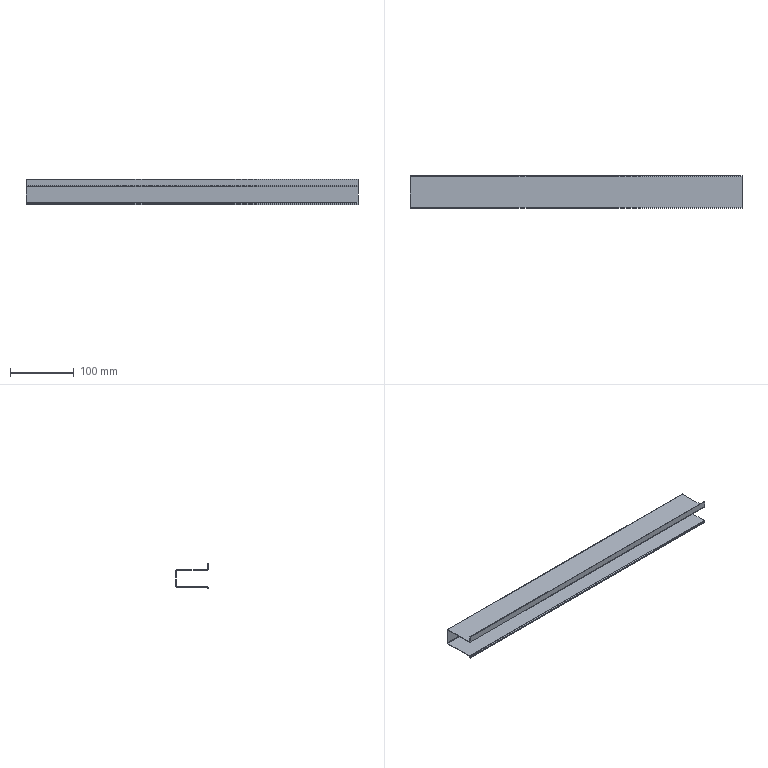Component | SolidWorks | ConnectingFlange-3 | 1 solid | 34 faces | box 520 x 50.74 x 40.07 mm | volume 52923 mm3 | plane 26 | cylinder 8 | commonest cylinder face diameters 2.946 x4 1.473 x4
STEP:
#1=COLOUR_RGB('',0.7922,0.8196,0.9333);
#2=FILL_AREA_STYLE_COLOUR('',#1);
#3=FILL_AREA_STYLE('',(#2));
#4=SURFACE_STYLE_FILL_AREA(#3);
#5=SURFACE_SIDE_STYLE('',(#4));
#6=SURFACE_STYLE_USAGE(.BOTH.,#5);
#7=PRESENTATION_STYLE_ASSIGNMENT((#6));
#8=CARTESIAN_POINT('',(-10.906,0.8454,2.992));
#9=VERTEX_POINT('',#8);
#10=CARTESIAN_POINT('',(-10.906,0.8454,2.963));
#11=VERTEX_POINT('',#10);
#12=CARTESIAN_POINT('',(-10.906,0.8454,2.992));
#13=DIRECTION('',(-0.,0.,-1.));
#14=VECTOR('',#13,39.37);
#15=LINE('',#12,#14);
#16=EDGE_CURVE('',#9,#11,#15,.T.);
#17=ORIENTED_EDGE('',*,*,#16,.F.);
#18=CARTESIAN_POINT('',(-10.906,2.727,2.992));
#19=VERTEX_POINT('',#18);
#20=CARTESIAN_POINT('',(-10.906,0.7874,2.992));
#21=DIRECTION('',(0.,-1.,0.));
#22=VECTOR('',#21,39.37);
#23=LINE('',#20,#22);
#24=EDGE_CURVE('',#19,#9,#23,.T.);
#25=ORIENTED_EDGE('',*,*,#24,.F.);
#26=CARTESIAN_POINT('',(-10.906,2.727,2.963));
#27=VERTEX_POINT('',#26);
#28=CARTESIAN_POINT('',(-10.906,2.727,2.963));
#29=DIRECTION('',(0.,0.,1.));
#30=VECTOR('',#29,39.37);
#31=LINE('',#28,#30);
#32=EDGE_CURVE('',#27,#19,#31,.T.);
#33=ORIENTED_EDGE('',*,*,#32,.F.);
#34=CARTESIAN_POINT('',(-10.906,0.7874,2.963));
#35=DIRECTION('',(0.,-1.,0.));
#36=VECTOR('',#35,39.37);
#37=LINE('',#34,#36);
#38=EDGE_CURVE('',#27,#11,#37,.T.);
#39=ORIENTED_EDGE('',*,*,#38,.T.);
#40=EDGE_LOOP('',(#17,#25,#33,#39));
#41=FACE_OUTER_BOUND('',#40,.T.);
#42=CARTESIAN_POINT('',(-10.906,0.7874,2.992));
#43=DIRECTION('',(1.,0.,0.));
#44=DIRECTION('',(-0.,1.,0.));
#45=AXIS2_PLACEMENT_3D('',#42,#43,#44);
#46=PLANE('',#45);
#47=ADVANCED_FACE('',(#41),#46,.F.);
#48=CARTESIAN_POINT('',(9.567,0.8454,2.992));
#49=VERTEX_POINT('',#48);
#50=CARTESIAN_POINT('',(9.567,0.8454,2.963));
#51=VERTEX_POINT('',#50);
#52=CARTESIAN_POINT('',(9.567,0.8454,2.992));
#53=DIRECTION('',(-0.,0.,-1.));
#54=VECTOR('',#53,39.37);
#55=LINE('',#52,#54);
#56=EDGE_CURVE('',#49,#51,#55,.T.);
#57=ORIENTED_EDGE('',*,*,#56,.T.);
#58=CARTESIAN_POINT('',(9.567,2.727,2.963));
#59=VERTEX_POINT('',#58);
#60=CARTESIAN_POINT('',(9.567,2.756,2.963));
#61=DIRECTION('',(-0.,1.,-0.));
#62=VECTOR('',#61,39.37);
#63=LINE('',#60,#62);
#64=EDGE_CURVE('',#51,#59,#63,.T.);
#65=ORIENTED_EDGE('',*,*,#64,.T.);
#66=CARTESIAN_POINT('',(9.567,2.727,2.992));
#67=VERTEX_POINT('',#66);
#68=CARTESIAN_POINT('',(9.567,2.727,2.992));
#69=DIRECTION('',(0.,0.,1.));
#70=VECTOR('',#69,39.37);
#71=LINE('',#68,#70);
#72=EDGE_CURVE('',#59,#67,#71,.T.);
#73=ORIENTED_EDGE('',*,*,#72,.T.);
#74=CARTESIAN_POINT('',(9.567,0.7874,2.992));
#75=DIRECTION('',(-0.,1.,-0.));
#76=VECTOR('',#75,39.37);
#77=LINE('',#74,#76);
#78=EDGE_CURVE('',#49,#67,#77,.T.);
#79=ORIENTED_EDGE('',*,*,#78,.F.);
#80=EDGE_LOOP('',(#57,#65,#73,#79));
#81=FACE_OUTER_BOUND('',#80,.T.);
#82=CARTESIAN_POINT('',(9.567,2.756,2.992));
#83=DIRECTION('',(-1.,-0.,-0.));
#84=DIRECTION('',(0.,-1.,-0.));
#85=AXIS2_PLACEMENT_3D('',#82,#83,#84);
#86=PLANE('',#85);
#87=ADVANCED_FACE('',(#81),#86,.F.);
#88=CARTESIAN_POINT('',(9.567,0.8454,2.992));
#89=DIRECTION('',(-1.,0.,0.));
#90=VECTOR('',#89,39.37);
#91=LINE('',#88,#90);
#92=EDGE_CURVE('',#49,#9,#91,.T.);
#93=ORIENTED_EDGE('',*,*,#92,.F.);
#94=ORIENTED_EDGE('',*,*,#78,.T.);
#95=CARTESIAN_POINT('',(9.567,2.727,2.992));
#96=DIRECTION('',(1.,-0.,0.));
#97=VECTOR('',#96,39.37);
#98=LINE('',#95,#97);
#99=EDGE_CURVE('',#19,#67,#98,.T.);
#100=ORIENTED_EDGE('',*,*,#99,.F.);
#101=ORIENTED_EDGE('',*,*,#24,.T.);
#102=EDGE_LOOP('',(#93,#94,#100,#101));
#103=FACE_OUTER_BOUND('',#102,.T.);
#104=CARTESIAN_POINT('',(-0.,0.7874,2.992));
#105=DIRECTION('',(-0.,-0.,-1.));
#106=DIRECTION('',(0.,-1.,0.));
#107=AXIS2_PLACEMENT_3D('',#104,#105,#106);
#108=PLANE('',#107);
#109=ADVANCED_FACE('',(#103),#108,.F.);
#110=ORIENTED_EDGE('',*,*,#64,.F.);
#111=CARTESIAN_POINT('',(9.567,0.8454,2.963));
#112=DIRECTION('',(-1.,0.,0.));
#113=VECTOR('',#112,39.37);
#114=LINE('',#111,#113);
#115=EDGE_CURVE('',#51,#11,#114,.T.);
#116=ORIENTED_EDGE('',*,*,#115,.T.);
#117=ORIENTED_EDGE('',*,*,#38,.F.);
#118=CARTESIAN_POINT('',(9.567,2.727,2.963));
#119=DIRECTION('',(-1.,0.,-0.));
#120=VECTOR('',#119,39.37);
#121=LINE('',#118,#120);
#122=EDGE_CURVE('',#59,#27,#121,.T.);
#123=ORIENTED_EDGE('',*,*,#122,.F.);
#124=EDGE_LOOP('',(#110,#116,#117,#123));
#125=FACE_OUTER_BOUND('',#124,.T.);
#126=CARTESIAN_POINT('',(-0.,0.7874,2.963));
#127=DIRECTION('',(-0.,-0.,-1.));
#128=DIRECTION('',(0.,-1.,0.));
#129=AXIS2_PLACEMENT_3D('',#126,#127,#128);
#130=PLANE('',#129);
#131=ADVANCED_FACE('',(#125),#130,.T.);
#132=CARTESIAN_POINT('',(-10.906,2.785,2.934));
#133=VERTEX_POINT('',#132);
#134=CARTESIAN_POINT('',(9.567,2.785,2.934));
#135=VERTEX_POINT('',#134);
#136=CARTESIAN_POINT('',(-10.906,2.785,2.934));
#137=DIRECTION('',(1.,-0.,-0.));
#138=VECTOR('',#137,39.37);
#139=LINE('',#136,#138);
#140=EDGE_CURVE('',#133,#135,#139,.T.);
#141=ORIENTED_EDGE('',*,*,#140,.T.);
#142=CARTESIAN_POINT('',(9.567,2.785,1.974));
#143=VERTEX_POINT('',#142);
#144=CARTESIAN_POINT('',(9.567,2.785,-19.895));
#145=DIRECTION('',(-0.,0.,-1.));
#146=VECTOR('',#145,39.37);
#147=LINE('',#144,#146);
#148=EDGE_CURVE('',#135,#143,#147,.T.);
#149=ORIENTED_EDGE('',*,*,#148,.T.);
#150=CARTESIAN_POINT('',(-10.906,2.785,1.974));
#151=VERTEX_POINT('',#150);
#152=CARTESIAN_POINT('',(10.906,2.785,1.974));
#153=DIRECTION('',(-1.,0.,0.));
#154=VECTOR('',#153,39.37);
#155=LINE('',#152,#154);
#156=EDGE_CURVE('',#143,#151,#155,.T.);
#157=ORIENTED_EDGE('',*,*,#156,.T.);
#158=CARTESIAN_POINT('',(-10.906,2.785,-19.895));
#159=DIRECTION('',(0.,-0.,1.));
#160=VECTOR('',#159,39.37);
#161=LINE('',#158,#160);
#162=EDGE_CURVE('',#151,#133,#161,.T.);
#163=ORIENTED_EDGE('',*,*,#162,.T.);
#164=EDGE_LOOP('',(#141,#149,#157,#163));
#165=FACE_OUTER_BOUND('',#164,.T.);
#166=CARTESIAN_POINT('',(-10.906,2.785,-19.895));
#167=DIRECTION('',(-0.,-1.,-0.));
#168=DIRECTION('',(1.,-0.,-0.));
#169=AXIS2_PLACEMENT_3D('',#166,#167,#168);
#170=PLANE('',#169);
#171=ADVANCED_FACE('',(#165),#170,.F.);
#172=CARTESIAN_POINT('',(9.567,2.756,2.934));
#173=VERTEX_POINT('',#172);
#174=CARTESIAN_POINT('',(9.567,2.756,1.974));
#175=VERTEX_POINT('',#174);
#176=CARTESIAN_POINT('',(9.567,2.756,-19.895));
#177=DIRECTION('',(-0.,0.,-1.));
#178=VECTOR('',#177,39.37);
#179=LINE('',#176,#178);
#180=EDGE_CURVE('',#173,#175,#179,.T.);
#181=ORIENTED_EDGE('',*,*,#180,.F.);
#182=CARTESIAN_POINT('',(-10.906,2.756,2.934));
#183=VERTEX_POINT('',#182);
#184=CARTESIAN_POINT('',(-10.906,2.756,2.934));
#185=DIRECTION('',(1.,-0.,-0.));
#186=VECTOR('',#185,39.37);
#187=LINE('',#184,#186);
#188=EDGE_CURVE('',#183,#173,#187,.T.);
#189=ORIENTED_EDGE('',*,*,#188,.F.);
#190=CARTESIAN_POINT('',(-10.906,2.756,1.974));
#191=VERTEX_POINT('',#190);
#192=CARTESIAN_POINT('',(-10.906,2.756,-19.895));
#193=DIRECTION('',(0.,-0.,1.));
#194=VECTOR('',#193,39.37);
#195=LINE('',#192,#194);
#196=EDGE_CURVE('',#191,#183,#195,.T.);
#197=ORIENTED_EDGE('',*,*,#196,.F.);
#198=CARTESIAN_POINT('',(10.906,2.756,1.974));
#199=DIRECTION('',(-1.,0.,0.));
#200=VECTOR('',#199,39.37);
#201=LINE('',#198,#200);
#202=EDGE_CURVE('',#175,#191,#201,.T.);
#203=ORIENTED_EDGE('',*,*,#202,.F.);
#204=EDGE_LOOP('',(#181,#189,#197,#203));
#205=FACE_OUTER_BOUND('',#204,.T.);
#206=CARTESIAN_POINT('',(-10.906,2.756,-19.895));
#207=DIRECTION('',(-0.,-1.,-0.));
#208=DIRECTION('',(1.,-0.,-0.));
#209=AXIS2_PLACEMENT_3D('',#206,#207,#208);
#210=PLANE('',#209);
#211=ADVANCED_FACE('',(#205),#210,.T.);
#212=ORIENTED_EDGE('',*,*,#196,.T.);
#213=CARTESIAN_POINT('',(-10.906,2.756,2.934));
#214=DIRECTION('',(-0.,1.,0.));
#215=VECTOR('',#214,39.37);
#216=LINE('',#213,#215);
#217=EDGE_CURVE('',#183,#133,#216,.T.);
#218=ORIENTED_EDGE('',*,*,#217,.T.);
#219=ORIENTED_EDGE('',*,*,#162,.F.);
#220=CARTESIAN_POINT('',(-10.906,2.756,1.974));
#221=DIRECTION('',(-0.,1.,0.));
#222=VECTOR('',#221,39.37);
#223=LINE('',#220,#222);
#224=EDGE_CURVE('',#191,#151,#223,.T.);
#225=ORIENTED_EDGE('',*,*,#224,.F.);
#226=EDGE_LOOP('',(#212,#218,#219,#225));
#227=FACE_OUTER_BOUND('',#226,.T.);
#228=CARTESIAN_POINT('',(-10.906,2.785,-19.895));
#229=DIRECTION('',(-1.,-0.,-0.));
#230=DIRECTION('',(0.,-1.,-0.));
#231=AXIS2_PLACEMENT_3D('',#228,#229,#230);
#232=PLANE('',#231);
#233=ADVANCED_FACE('',(#227),#232,.T.);
#234=CARTESIAN_POINT('',(9.567,2.756,2.934));
#235=DIRECTION('',(-0.,1.,0.));
#236=VECTOR('',#235,39.37);
#237=LINE('',#234,#236);
#238=EDGE_CURVE('',#173,#135,#237,.T.);
#239=ORIENTED_EDGE('',*,*,#238,.F.);
#240=ORIENTED_EDGE('',*,*,#180,.T.);
#241=CARTESIAN_POINT('',(9.567,2.727,1.945));
#242=VERTEX_POINT('',#241);
#243=CARTESIAN_POINT('',(9.567,2.727,1.974));
#244=DIRECTION('',(1.,-0.,-0.));
#245=DIRECTION('',(0.,-1.,0.));
#246=AXIS2_PLACEMENT_3D('',#243,#244,#245);
#247=CIRCLE('',#246,0.029);
#248=EDGE_CURVE('',#242,#175,#247,.T.);
#249=ORIENTED_EDGE('',*,*,#248,.F.);
#250=CARTESIAN_POINT('',(9.567,0.8454,1.945));
#251=VERTEX_POINT('',#250);
#252=CARTESIAN_POINT('',(9.567,0.7874,1.945));
#253=DIRECTION('',(0.,-1.,-0.));
#254=VECTOR('',#253,39.37);
#255=LINE('',#252,#254);
#256=EDGE_CURVE('',#242,#251,#255,.T.);
#257=ORIENTED_EDGE('',*,*,#256,.T.);
#258=CARTESIAN_POINT('',(9.567,0.7874,1.887));
#259=VERTEX_POINT('',#258);
#260=CARTESIAN_POINT('',(9.567,0.8454,1.887));
#261=DIRECTION('',(1.,-0.,-0.));
#262=DIRECTION('',(0.,-1.,-0.));
#263=AXIS2_PLACEMENT_3D('',#260,#261,#262);
#264=CIRCLE('',#263,0.058);
#265=EDGE_CURVE('',#251,#259,#264,.T.);
#266=ORIENTED_EDGE('',*,*,#265,.T.);
#267=CARTESIAN_POINT('',(9.567,0.7874,1.819));
#268=VERTEX_POINT('',#267);
#269=CARTESIAN_POINT('',(9.567,0.7874,-4.553));
#270=DIRECTION('',(0.,-0.,1.));
#271=VECTOR('',#270,39.37);
#272=LINE('',#269,#271);
#273=EDGE_CURVE('',#268,#259,#272,.T.);
#274=ORIENTED_EDGE('',*,*,#273,.F.);
#275=CARTESIAN_POINT('',(9.567,0.8164,1.819));
#276=VERTEX_POINT('',#275);
#277=CARTESIAN_POINT('',(9.567,0.7874,1.819));
#278=DIRECTION('',(0.,-1.,-0.));
#279=VECTOR('',#278,39.37);
#280=LINE('',#277,#279);
#281=EDGE_CURVE('',#276,#268,#280,.T.);
#282=ORIENTED_EDGE('',*,*,#281,.F.);
#283=CARTESIAN_POINT('',(9.567,0.8164,1.887));
#284=VERTEX_POINT('',#283);
#285=CARTESIAN_POINT('',(9.567,0.8164,0.));
#286=DIRECTION('',(0.,-0.,1.));
#287=VECTOR('',#286,39.37);
#288=LINE('',#285,#287);
#289=EDGE_CURVE('',#276,#284,#288,.T.);
#290=ORIENTED_EDGE('',*,*,#289,.T.);
#291=CARTESIAN_POINT('',(9.567,0.8454,1.916));
#292=VERTEX_POINT('',#291);
#293=CARTESIAN_POINT('',(9.567,0.8454,1.887));
#294=DIRECTION('',(1.,-0.,-0.));
#295=DIRECTION('',(0.,-1.,-0.));
#296=AXIS2_PLACEMENT_3D('',#293,#294,#295);
#297=CIRCLE('',#296,0.029);
#298=EDGE_CURVE('',#292,#284,#297,.T.);
#299=ORIENTED_EDGE('',*,*,#298,.F.);
#300=CARTESIAN_POINT('',(9.567,2.727,1.916));
#301=VERTEX_POINT('',#300);
#302=CARTESIAN_POINT('',(9.567,0.7874,1.916));
#303=DIRECTION('',(0.,-1.,-0.));
#304=VECTOR('',#303,39.37);
#305=LINE('',#302,#304);
#306=EDGE_CURVE('',#301,#292,#305,.T.);
#307=ORIENTED_EDGE('',*,*,#306,.F.);
#308=CARTESIAN_POINT('',(9.567,2.727,1.974));
#309=DIRECTION('',(1.,-0.,-0.));
#310=DIRECTION('',(0.,-1.,0.));
#311=AXIS2_PLACEMENT_3D('',#308,#309,#310);
#312=CIRCLE('',#311,0.058);
#313=EDGE_CURVE('',#301,#143,#312,.T.);
#314=ORIENTED_EDGE('',*,*,#313,.T.);
#315=ORIENTED_EDGE('',*,*,#148,.F.);
#316=EDGE_LOOP('',(#239,#240,#249,#257,#266,#274,#282,#290,#299,#307,#314,#315));
#317=FACE_OUTER_BOUND('',#316,.T.);
#318=CARTESIAN_POINT('',(9.567,0.7874,-4.553));
#319=DIRECTION('',(-1.,-0.,-0.));
#320=DIRECTION('',(0.,-1.,-0.));
#321=AXIS2_PLACEMENT_3D('',#318,#319,#320);
#322=PLANE('',#321);
#323=ADVANCED_FACE('',(#317),#322,.F.);
#324=CARTESIAN_POINT('',(-10.906,0.8454,1.916));
#325=VERTEX_POINT('',#324);
#326=CARTESIAN_POINT('',(-10.906,0.8454,1.945));
#327=VERTEX_POINT('',#326);
#328=CARTESIAN_POINT('',(-10.906,0.8454,1.916));
#329=DIRECTION('',(0.,-0.,1.));
#330=VECTOR('',#329,39.37);
#331=LINE('',#328,#330);
#332=EDGE_CURVE('',#325,#327,#331,.T.);
#333=ORIENTED_EDGE('',*,*,#332,.T.);
#334=CARTESIAN_POINT('',(-10.906,2.727,1.945));
#335=VERTEX_POINT('',#334);
#336=CARTESIAN_POINT('',(-10.906,2.756,1.945));
#337=DIRECTION('',(-0.,1.,0.));
#338=VECTOR('',#337,39.37);
#339=LINE('',#336,#338);
#340=EDGE_CURVE('',#327,#335,#339,.T.);
#341=ORIENTED_EDGE('',*,*,#340,.T.);
#342=CARTESIAN_POINT('',(-10.906,2.727,1.916));
#343=VERTEX_POINT('',#342);
#344=CARTESIAN_POINT('',(-10.906,2.727,1.916));
#345=DIRECTION('',(0.,0.,-1.));
#346=VECTOR('',#345,39.37);
#347=LINE('',#344,#346);
#348=EDGE_CURVE('',#335,#343,#347,.T.);
#349=ORIENTED_EDGE('',*,*,#348,.T.);
#350=CARTESIAN_POINT('',(-10.906,0.7874,1.916));
#351=DIRECTION('',(-0.,1.,0.));
#352=VECTOR('',#351,39.37);
#353=LINE('',#350,#352);
#354=EDGE_CURVE('',#325,#343,#353,.T.);
#355=ORIENTED_EDGE('',*,*,#354,.F.);
#356=EDGE_LOOP('',(#333,#341,#349,#355));
#357=FACE_OUTER_BOUND('',#356,.T.);
#358=CARTESIAN_POINT('',(-10.906,2.756,1.916));
#359=DIRECTION('',(1.,-0.,0.));
#360=DIRECTION('',(0.,0.,-1.));
#361=AXIS2_PLACEMENT_3D('',#358,#359,#360);
#362=PLANE('',#361);
#363=ADVANCED_FACE('',(#357),#362,.F.);
#364=CARTESIAN_POINT('',(-10.906,2.727,1.916));
#365=DIRECTION('',(-1.,0.,-0.));
#366=VECTOR('',#365,39.37);
#367=LINE('',#364,#366);
#368=EDGE_CURVE('',#301,#343,#367,.T.);
#369=ORIENTED_EDGE('',*,*,#368,.F.);
#370=ORIENTED_EDGE('',*,*,#306,.T.);
#371=CARTESIAN_POINT('',(-10.906,0.8454,1.916));
#372=DIRECTION('',(1.,-0.,-0.));
#373=VECTOR('',#372,39.37);
#374=LINE('',#371,#373);
#375=EDGE_CURVE('',#325,#292,#374,.T.);
#376=ORIENTED_EDGE('',*,*,#375,.F.);
#377=ORIENTED_EDGE('',*,*,#354,.T.);
#378=EDGE_LOOP('',(#369,#370,#376,#377));
#379=FACE_OUTER_BOUND('',#378,.T.);
#380=CARTESIAN_POINT('',(-0.,0.7874,1.916));
#381=DIRECTION('',(-0.,-0.,1.));
#382=DIRECTION('',(-0.,1.,0.));
#383=AXIS2_PLACEMENT_3D('',#380,#381,#382);
#384=PLANE('',#383);
#385=ADVANCED_FACE('',(#379),#384,.F.);
#386=ORIENTED_EDGE('',*,*,#256,.F.);
#387=CARTESIAN_POINT('',(-10.906,2.727,1.945));
#388=DIRECTION('',(1.,-0.,0.));
#389=VECTOR('',#388,39.37);
#390=LINE('',#387,#389);
#391=EDGE_CURVE('',#335,#242,#390,.T.);
#392=ORIENTED_EDGE('',*,*,#391,.F.);
#393=ORIENTED_EDGE('',*,*,#340,.F.);
#394=CARTESIAN_POINT('',(-10.906,0.8454,1.945));
#395=DIRECTION('',(1.,-0.,-0.));
#396=VECTOR('',#395,39.37);
#397=LINE('',#394,#396);
#398=EDGE_CURVE('',#327,#251,#397,.T.);
#399=ORIENTED_EDGE('',*,*,#398,.T.);
#400=EDGE_LOOP('',(#386,#392,#393,#399));
#401=FACE_OUTER_BOUND('',#400,.T.);
#402=CARTESIAN_POINT('',(-0.,0.7874,1.945));
#403=DIRECTION('',(-0.,-0.,1.));
#404=DIRECTION('',(-0.,1.,0.));
#405=AXIS2_PLACEMENT_3D('',#402,#403,#404);
#406=PLANE('',#405);
#407=ADVANCED_FACE('',(#401),#406,.T.);
#408=ORIENTED_EDGE('',*,*,#348,.F.);
#409=CARTESIAN_POINT('',(-10.906,2.727,1.974));
#410=DIRECTION('',(-1.,0.,0.));
#411=DIRECTION('',(0.,1.,-0.));
#412=AXIS2_PLACEMENT_3D('',#409,#410,#411);
#413=CIRCLE('',#412,0.029);
#414=EDGE_CURVE('',#191,#335,#413,.T.);
#415=ORIENTED_EDGE('',*,*,#414,.F.);
#416=ORIENTED_EDGE('',*,*,#224,.T.);
#417=CARTESIAN_POINT('',(-10.906,2.727,1.974));
#418=DIRECTION('',(-1.,0.,0.));
#419=DIRECTION('',(0.,1.,0.));
#420=AXIS2_PLACEMENT_3D('',#417,#418,#419);
#421=CIRCLE('',#420,0.058);
#422=EDGE_CURVE('',#151,#343,#421,.T.);
#423=ORIENTED_EDGE('',*,*,#422,.T.);
#424=EDGE_LOOP('',(#408,#415,#416,#423));
#425=FACE_OUTER_BOUND('',#424,.T.);
#426=CARTESIAN_POINT('',(-10.906,2.727,1.974));
#427=DIRECTION('',(-1.,-0.,-0.));
#428=DIRECTION('',(0.,-1.,-0.));
#429=AXIS2_PLACEMENT_3D('',#426,#427,#428);
#430=PLANE('',#429);
#431=ADVANCED_FACE('',(#425),#430,.T.);
#432=ORIENTED_EDGE('',*,*,#313,.F.);
#433=ORIENTED_EDGE('',*,*,#368,.T.);
#434=ORIENTED_EDGE('',*,*,#422,.F.);
#435=ORIENTED_EDGE('',*,*,#156,.F.);
#436=EDGE_LOOP('',(#432,#433,#434,#435));
#437=FACE_OUTER_BOUND('',#436,.T.);
#438=CARTESIAN_POINT('',(10.906,2.727,1.974));
#439=DIRECTION('',(1.,-0.,-0.));
#440=DIRECTION('',(0.,0.,-1.));
#441=AXIS2_PLACEMENT_3D('',#438,#439,#440);
#442=CYLINDRICAL_SURFACE('',#441,0.058);
#443=ADVANCED_FACE('',(#437),#442,.T.);
#444=ORIENTED_EDGE('',*,*,#391,.T.);
#445=ORIENTED_EDGE('',*,*,#248,.T.);
#446=ORIENTED_EDGE('',*,*,#202,.T.);
#447=ORIENTED_EDGE('',*,*,#414,.T.);
#448=EDGE_LOOP('',(#444,#445,#446,#447));
#449=FACE_OUTER_BOUND('',#448,.T.);
#450=CARTESIAN_POINT('',(10.906,2.727,1.974));
#451=DIRECTION('',(1.,-0.,-0.));
#452=DIRECTION('',(0.,0.,-1.));
#453=AXIS2_PLACEMENT_3D('',#450,#451,#452);
#454=CYLINDRICAL_SURFACE('',#453,0.029);
#455=ADVANCED_FACE('',(#449),#454,.F.);
#456=CARTESIAN_POINT('',(-10.906,0.8164,1.887));
#457=VERTEX_POINT('',#456);
#458=CARTESIAN_POINT('',(-10.906,0.8454,1.887));
#459=DIRECTION('',(-1.,0.,0.));
#460=DIRECTION('',(0.,-1.,0.));
#461=AXIS2_PLACEMENT_3D('',#458,#459,#460);
#462=CIRCLE('',#461,0.029);
#463=EDGE_CURVE('',#457,#325,#462,.T.);
#464=ORIENTED_EDGE('',*,*,#463,.F.);
#465=CARTESIAN_POINT('',(-10.906,0.7874,1.887));
#466=VERTEX_POINT('',#465);
#467=CARTESIAN_POINT('',(-10.906,0.8164,1.887));
#468=DIRECTION('',(0.,-1.,0.));
#469=VECTOR('',#468,39.37);
#470=LINE('',#467,#469);
#471=EDGE_CURVE('',#457,#466,#470,.T.);
#472=ORIENTED_EDGE('',*,*,#471,.T.);
#473=CARTESIAN_POINT('',(-10.906,0.8454,1.887));
#474=DIRECTION('',(-1.,0.,0.));
#475=DIRECTION('',(0.,-1.,0.));
#476=AXIS2_PLACEMENT_3D('',#473,#474,#475);
#477=CIRCLE('',#476,0.058);
#478=EDGE_CURVE('',#466,#327,#477,.T.);
#479=ORIENTED_EDGE('',*,*,#478,.T.);
#480=ORIENTED_EDGE('',*,*,#332,.F.);
#481=EDGE_LOOP('',(#464,#472,#479,#480));
#482=FACE_OUTER_BOUND('',#481,.T.);
#483=CARTESIAN_POINT('',(-10.906,0.8454,1.887));
#484=DIRECTION('',(1.,-0.,-0.));
#485=DIRECTION('',(0.,1.,0.));
#486=AXIS2_PLACEMENT_3D('',#483,#484,#485);
#487=PLANE('',#486);
#488=ADVANCED_FACE('',(#482),#487,.F.);
#489=ORIENTED_EDGE('',*,*,#265,.F.);
#490=ORIENTED_EDGE('',*,*,#398,.F.);
#491=ORIENTED_EDGE('',*,*,#478,.F.);
#492=CARTESIAN_POINT('',(10.906,0.7874,1.887));
#493=DIRECTION('',(1.,-0.,0.));
#494=VECTOR('',#493,39.37);
#495=LINE('',#492,#494);
#496=EDGE_CURVE('',#466,#259,#495,.T.);
#497=ORIENTED_EDGE('',*,*,#496,.T.);
#498=EDGE_LOOP('',(#489,#490,#491,#497));
#499=FACE_OUTER_BOUND('',#498,.T.);
#500=CARTESIAN_POINT('',(-10.906,0.8454,1.887));
#501=DIRECTION('',(-1.,0.,0.));
#502=DIRECTION('',(0.,-1.,0.));
#503=AXIS2_PLACEMENT_3D('',#500,#501,#502);
#504=CYLINDRICAL_SURFACE('',#503,0.058);
#505=ADVANCED_FACE('',(#499),#504,.T.);
#506=ORIENTED_EDGE('',*,*,#375,.T.);
#507=ORIENTED_EDGE('',*,*,#298,.T.);
#508=CARTESIAN_POINT('',(10.906,0.8164,1.887));
#509=DIRECTION('',(-1.,0.,-0.));
#510=VECTOR('',#509,39.37);
#511=LINE('',#508,#510);
#512=EDGE_CURVE('',#284,#457,#511,.T.);
#513=ORIENTED_EDGE('',*,*,#512,.T.);
#514=ORIENTED_EDGE('',*,*,#463,.T.);
#515=EDGE_LOOP('',(#506,#507,#513,#514));
#516=FACE_OUTER_BOUND('',#515,.T.);
#517=CARTESIAN_POINT('',(-10.906,0.8454,1.887));
#518=DIRECTION('',(-1.,0.,0.));
#519=DIRECTION('',(0.,-1.,0.));
#520=AXIS2_PLACEMENT_3D('',#517,#518,#519);
#521=CYLINDRICAL_SURFACE('',#520,0.029);
#522=ADVANCED_FACE('',(#516),#521,.F.);
#523=ORIENTED_EDGE('',*,*,#471,.F.);
#524=CARTESIAN_POINT('',(-10.906,0.8164,1.819));
#525=VERTEX_POINT('',#524);
#526=CARTESIAN_POINT('',(-10.906,0.8164,1.819));
#527=DIRECTION('',(-0.,0.,-1.));
#528=VECTOR('',#527,39.37);
#529=LINE('',#526,#528);
#530=EDGE_CURVE('',#457,#525,#529,.T.);
#531=ORIENTED_EDGE('',*,*,#530,.T.);
#532=CARTESIAN_POINT('',(-10.906,0.7874,1.819));
#533=VERTEX_POINT('',#532);
#534=CARTESIAN_POINT('',(-10.906,0.7874,1.819));
#535=DIRECTION('',(-0.,1.,0.));
#536=VECTOR('',#535,39.37);
#537=LINE('',#534,#536);
#538=EDGE_CURVE('',#533,#525,#537,.T.);
#539=ORIENTED_EDGE('',*,*,#538,.F.);
#540=CARTESIAN_POINT('',(-10.906,0.7874,0.));
#541=DIRECTION('',(-0.,0.,-1.));
#542=VECTOR('',#541,39.37);
#543=LINE('',#540,#542);
#544=EDGE_CURVE('',#466,#533,#543,.T.);
#545=ORIENTED_EDGE('',*,*,#544,.F.);
#546=EDGE_LOOP('',(#523,#531,#539,#545));
#547=FACE_OUTER_BOUND('',#546,.T.);
#548=CARTESIAN_POINT('',(-10.906,0.7874,1.819));
#549=DIRECTION('',(1.,0.,0.));
#550=DIRECTION('',(-0.,1.,0.));
#551=AXIS2_PLACEMENT_3D('',#548,#549,#550);
#552=PLANE('',#551);
#553=ADVANCED_FACE('',(#547),#552,.F.);
#554=CARTESIAN_POINT('',(-0.,0.7874,1.819));
#555=DIRECTION('',(1.,-0.,0.));
#556=VECTOR('',#555,39.37);
#557=LINE('',#554,#556);
#558=EDGE_CURVE('',#533,#268,#557,.T.);
#559=ORIENTED_EDGE('',*,*,#558,.T.);
#560=ORIENTED_EDGE('',*,*,#273,.T.);
#561=ORIENTED_EDGE('',*,*,#496,.F.);
#562=ORIENTED_EDGE('',*,*,#544,.T.);
#563=EDGE_LOOP('',(#559,#560,#561,#562));
#564=FACE_OUTER_BOUND('',#563,.T.);
#565=CARTESIAN_POINT('',(-0.,0.7874,0.));
#566=DIRECTION('',(-0.,1.,0.));
#567=DIRECTION('',(-0.,0.,-1.));
#568=AXIS2_PLACEMENT_3D('',#565,#566,#567);
#569=PLANE('',#568);
#570=ADVANCED_FACE('',(#564),#569,.F.);
#571=ORIENTED_EDGE('',*,*,#289,.F.);
#572=CARTESIAN_POINT('',(10.906,0.8164,1.819));
#573=DIRECTION('',(1.,-0.,0.));
#574=VECTOR('',#573,39.37);
#575=LINE('',#572,#574);
#576=EDGE_CURVE('',#525,#276,#575,.T.);
#577=ORIENTED_EDGE('',*,*,#576,.F.);
#578=ORIENTED_EDGE('',*,*,#530,.F.);
#579=ORIENTED_EDGE('',*,*,#512,.F.);
#580=EDGE_LOOP('',(#571,#577,#578,#579));
#581=FACE_OUTER_BOUND('',#580,.T.);
#582=CARTESIAN_POINT('',(-0.,0.8164,0.));
#583=DIRECTION('',(-0.,1.,0.));
#584=DIRECTION('',(-0.,0.,-1.));
#585=AXIS2_PLACEMENT_3D('',#582,#583,#584);
#586=PLANE('',#585);
#587=ADVANCED_FACE('',(#581),#586,.T.);
#588=ORIENTED_EDGE('',*,*,#576,.T.);
#589=ORIENTED_EDGE('',*,*,#281,.T.);
#590=ORIENTED_EDGE('',*,*,#558,.F.);
#591=ORIENTED_EDGE('',*,*,#538,.T.);
#592=EDGE_LOOP('',(#588,#589,#590,#591));
#593=FACE_OUTER_BOUND('',#592,.T.);
#594=CARTESIAN_POINT('',(10.906,0.7874,1.819));
#595=DIRECTION('',(-0.,-0.,1.));
#596=DIRECTION('',(1.,-0.,0.));
#597=AXIS2_PLACEMENT_3D('',#594,#595,#596);
#598=PLANE('',#597);
#599=ADVANCED_FACE('',(#593),#598,.F.);
#600=ORIENTED_EDGE('',*,*,#72,.F.);
#601=CARTESIAN_POINT('',(9.567,2.727,2.934));
#602=DIRECTION('',(1.,-0.,-0.));
#603=DIRECTION('',(0.,-1.,0.));
#604=AXIS2_PLACEMENT_3D('',#601,#602,#603);
#605=CIRCLE('',#604,0.029);
#606=EDGE_CURVE('',#173,#59,#605,.T.);
#607=ORIENTED_EDGE('',*,*,#606,.F.);
#608=ORIENTED_EDGE('',*,*,#238,.T.);
#609=CARTESIAN_POINT('',(9.567,2.727,2.934));
#610=DIRECTION('',(1.,-0.,-0.));
#611=DIRECTION('',(0.,-1.,0.));
#612=AXIS2_PLACEMENT_3D('',#609,#610,#611);
#613=CIRCLE('',#612,0.058);
#614=EDGE_CURVE('',#135,#67,#613,.T.);
#615=ORIENTED_EDGE('',*,*,#614,.T.);
#616=EDGE_LOOP('',(#600,#607,#608,#615));
#617=FACE_OUTER_BOUND('',#616,.T.);
#618=CARTESIAN_POINT('',(9.567,2.727,2.934));
#619=DIRECTION('',(1.,0.,0.));
#620=DIRECTION('',(-0.,1.,0.));
#621=AXIS2_PLACEMENT_3D('',#618,#619,#620);
#622=PLANE('',#621);
#623=ADVANCED_FACE('',(#617),#622,.T.);
#624=CARTESIAN_POINT('',(-10.906,2.727,2.934));
#625=DIRECTION('',(-1.,0.,0.));
#626=DIRECTION('',(0.,-1.,0.));
#627=AXIS2_PLACEMENT_3D('',#624,#625,#626);
#628=CIRCLE('',#627,0.029);
#629=EDGE_CURVE('',#27,#183,#628,.T.);
#630=ORIENTED_EDGE('',*,*,#629,.F.);
#631=ORIENTED_EDGE('',*,*,#32,.T.);
#632=CARTESIAN_POINT('',(-10.906,2.727,2.934));
#633=DIRECTION('',(-1.,0.,0.));
#634=DIRECTION('',(0.,-1.,0.));
#635=AXIS2_PLACEMENT_3D('',#632,#633,#634);
#636=CIRCLE('',#635,0.058);
#637=EDGE_CURVE('',#19,#133,#636,.T.);
#638=ORIENTED_EDGE('',*,*,#637,.T.);
#639=ORIENTED_EDGE('',*,*,#217,.F.);
#640=EDGE_LOOP('',(#630,#631,#638,#639));
#641=FACE_OUTER_BOUND('',#640,.T.);
#642=CARTESIAN_POINT('',(-10.906,2.727,2.934));
#643=DIRECTION('',(1.,0.,0.));
#644=DIRECTION('',(-0.,1.,0.));
#645=AXIS2_PLACEMENT_3D('',#642,#643,#644);
#646=PLANE('',#645);
#647=ADVANCED_FACE('',(#641),#646,.F.);
#648=ORIENTED_EDGE('',*,*,#140,.F.);
#649=ORIENTED_EDGE('',*,*,#637,.F.);
#650=ORIENTED_EDGE('',*,*,#99,.T.);
#651=ORIENTED_EDGE('',*,*,#614,.F.);
#652=EDGE_LOOP('',(#648,#649,#650,#651));
#653=FACE_OUTER_BOUND('',#652,.T.);
#654=CARTESIAN_POINT('',(-10.906,2.727,2.934));
#655=DIRECTION('',(-1.,0.,0.));
#656=DIRECTION('',(0.,0.,1.));
#657=AXIS2_PLACEMENT_3D('',#654,#655,#656);
#658=CYLINDRICAL_SURFACE('',#657,0.058);
#659=ADVANCED_FACE('',(#653),#658,.T.);
#660=ORIENTED_EDGE('',*,*,#188,.T.);
#661=ORIENTED_EDGE('',*,*,#606,.T.);
#662=ORIENTED_EDGE('',*,*,#122,.T.);
#663=ORIENTED_EDGE('',*,*,#629,.T.);
#664=EDGE_LOOP('',(#660,#661,#662,#663));
#665=FACE_OUTER_BOUND('',#664,.T.);
#666=CARTESIAN_POINT('',(-10.906,2.727,2.934));
#667=DIRECTION('',(-1.,0.,0.));
#668=DIRECTION('',(0.,0.,1.));
#669=AXIS2_PLACEMENT_3D('',#666,#667,#668);
#670=CYLINDRICAL_SURFACE('',#669,0.029);
#671=ADVANCED_FACE('',(#665),#670,.F.);
#672=CARTESIAN_POINT('',(-10.906,0.8164,3.021));
#673=VERTEX_POINT('',#672);
#674=CARTESIAN_POINT('',(-10.906,0.7874,3.021));
#675=VERTEX_POINT('',#674);
#676=CARTESIAN_POINT('',(-10.906,0.7874,3.021));
#677=DIRECTION('',(0.,-1.,0.));
#678=VECTOR('',#677,39.37);
#679=LINE('',#676,#678);
#680=EDGE_CURVE('',#673,#675,#679,.T.);
#681=ORIENTED_EDGE('',*,*,#680,.F.);
#682=CARTESIAN_POINT('',(-10.906,0.8454,3.021));
#683=DIRECTION('',(-1.,0.,0.));
#684=DIRECTION('',(0.,1.,0.));
#685=AXIS2_PLACEMENT_3D('',#682,#683,#684);
#686=CIRCLE('',#685,0.029);
#687=EDGE_CURVE('',#9,#673,#686,.T.);
#688=ORIENTED_EDGE('',*,*,#687,.F.);
#689=ORIENTED_EDGE('',*,*,#16,.T.);
#690=CARTESIAN_POINT('',(-10.906,0.8454,3.021));
#691=DIRECTION('',(-1.,0.,0.));
#692=DIRECTION('',(0.,1.,0.));
#693=AXIS2_PLACEMENT_3D('',#690,#691,#692);
#694=CIRCLE('',#693,0.058);
#695=EDGE_CURVE('',#11,#675,#694,.T.);
#696=ORIENTED_EDGE('',*,*,#695,.T.);
#697=EDGE_LOOP('',(#681,#688,#689,#696));
#698=FACE_OUTER_BOUND('',#697,.T.);
#699=CARTESIAN_POINT('',(-10.906,0.8454,3.021));
#700=DIRECTION('',(-1.,0.,0.));
#701=DIRECTION('',(-0.,-1.,-0.));
#702=AXIS2_PLACEMENT_3D('',#699,#700,#701);
#703=PLANE('',#702);
#704=ADVANCED_FACE('',(#698),#703,.T.);
#705=CARTESIAN_POINT('',(9.567,0.8164,3.021));
#706=VERTEX_POINT('',#705);
#707=CARTESIAN_POINT('',(9.567,0.8454,3.021));
#708=DIRECTION('',(1.,-0.,-0.));
#709=DIRECTION('',(0.,1.,0.));
#710=AXIS2_PLACEMENT_3D('',#707,#708,#709);
#711=CIRCLE('',#710,0.029);
#712=EDGE_CURVE('',#706,#49,#711,.T.);
#713=ORIENTED_EDGE('',*,*,#712,.F.);
#714=CARTESIAN_POINT('',(9.567,0.7874,3.021));
#715=VERTEX_POINT('',#714);
#716=CARTESIAN_POINT('',(9.567,0.8164,3.021));
#717=DIRECTION('',(0.,-1.,0.));
#718=VECTOR('',#717,39.37);
#719=LINE('',#716,#718);
#720=EDGE_CURVE('',#706,#715,#719,.T.);
#721=ORIENTED_EDGE('',*,*,#720,.T.);
#722=CARTESIAN_POINT('',(9.567,0.8454,3.021));
#723=DIRECTION('',(1.,-0.,-0.));
#724=DIRECTION('',(0.,1.,0.));
#725=AXIS2_PLACEMENT_3D('',#722,#723,#724);
#726=CIRCLE('',#725,0.058);
#727=EDGE_CURVE('',#715,#51,#726,.T.);
#728=ORIENTED_EDGE('',*,*,#727,.T.);
#729=ORIENTED_EDGE('',*,*,#56,.F.);
#730=EDGE_LOOP('',(#713,#721,#728,#729));
#731=FACE_OUTER_BOUND('',#730,.T.);
#732=CARTESIAN_POINT('',(9.567,0.8454,3.021));
#733=DIRECTION('',(-1.,0.,0.));
#734=DIRECTION('',(-0.,-1.,-0.));
#735=AXIS2_PLACEMENT_3D('',#732,#733,#734);
#736=PLANE('',#735);
#737=ADVANCED_FACE('',(#731),#736,.F.);
#738=ORIENTED_EDGE('',*,*,#115,.F.);
#739=ORIENTED_EDGE('',*,*,#727,.F.);
#740=CARTESIAN_POINT('',(-10.906,0.7874,3.021));
#741=DIRECTION('',(-1.,0.,0.));
#742=VECTOR('',#741,39.37);
#743=LINE('',#740,#742);
#744=EDGE_CURVE('',#715,#675,#743,.T.);
#745=ORIENTED_EDGE('',*,*,#744,.T.);
#746=ORIENTED_EDGE('',*,*,#695,.F.);
#747=EDGE_LOOP('',(#738,#739,#745,#746));
#748=FACE_OUTER_BOUND('',#747,.T.);
#749=CARTESIAN_POINT('',(9.567,0.8454,3.021));
#750=DIRECTION('',(1.,-0.,-0.));
#751=DIRECTION('',(0.,-1.,0.));
#752=AXIS2_PLACEMENT_3D('',#749,#750,#751);
#753=CYLINDRICAL_SURFACE('',#752,0.058);
#754=ADVANCED_FACE('',(#748),#753,.T.);
#755=ORIENTED_EDGE('',*,*,#92,.T.);
#756=ORIENTED_EDGE('',*,*,#687,.T.);
#757=CARTESIAN_POINT('',(-10.906,0.8164,3.021));
#758=DIRECTION('',(1.,-0.,-0.));
#759=VECTOR('',#758,39.37);
#760=LINE('',#757,#759);
#761=EDGE_CURVE('',#673,#706,#760,.T.);
#762=ORIENTED_EDGE('',*,*,#761,.T.);
#763=ORIENTED_EDGE('',*,*,#712,.T.);
#764=EDGE_LOOP('',(#755,#756,#762,#763));
#765=FACE_OUTER_BOUND('',#764,.T.);
#766=CARTESIAN_POINT('',(9.567,0.8454,3.021));
#767=DIRECTION('',(1.,-0.,-0.));
#768=DIRECTION('',(0.,-1.,0.));
#769=AXIS2_PLACEMENT_3D('',#766,#767,#768);
#770=CYLINDRICAL_SURFACE('',#769,0.029);
#771=ADVANCED_FACE('',(#765),#770,.F.);
#772=ORIENTED_EDGE('',*,*,#720,.F.);
#773=CARTESIAN_POINT('',(9.567,0.8164,3.396));
#774=VERTEX_POINT('',#773);
#775=CARTESIAN_POINT('',(9.567,0.8164,3.396));
#776=DIRECTION('',(0.,0.,1.));
#777=VECTOR('',#776,39.37);
#778=LINE('',#775,#777);
#779=EDGE_CURVE('',#706,#774,#778,.T.);
#780=ORIENTED_EDGE('',*,*,#779,.T.);
#781=CARTESIAN_POINT('',(9.567,0.7874,3.396));
#782=VERTEX_POINT('',#781);
#783=CARTESIAN_POINT('',(9.567,0.7874,3.396));
#784=DIRECTION('',(-0.,1.,0.));
#785=VECTOR('',#784,39.37);
#786=LINE('',#783,#785);
#787=EDGE_CURVE('',#782,#774,#786,.T.);
#788=ORIENTED_EDGE('',*,*,#787,.F.);
#789=CARTESIAN_POINT('',(9.567,0.7874,0.));
#790=DIRECTION('',(0.,0.,1.));
#791=VECTOR('',#790,39.37);
#792=LINE('',#789,#791);
#793=EDGE_CURVE('',#715,#782,#792,.T.);
#794=ORIENTED_EDGE('',*,*,#793,.F.);
#795=EDGE_LOOP('',(#772,#780,#788,#794));
#796=FACE_OUTER_BOUND('',#795,.T.);
#797=CARTESIAN_POINT('',(9.567,0.7874,3.396));
#798=DIRECTION('',(-1.,-0.,-0.));
#799=DIRECTION('',(0.,-1.,-0.));
#800=AXIS2_PLACEMENT_3D('',#797,#798,#799);
#801=PLANE('',#800);
#802=ADVANCED_FACE('',(#796),#801,.F.);
#803=ORIENTED_EDGE('',*,*,#680,.T.);
#804=CARTESIAN_POINT('',(-10.906,0.7874,3.396));
#805=VERTEX_POINT('',#804);
#806=CARTESIAN_POINT('',(-10.906,0.7874,0.));
#807=DIRECTION('',(-0.,-0.,-1.));
#808=VECTOR('',#807,39.37);
#809=LINE('',#806,#808);
#810=EDGE_CURVE('',#805,#675,#809,.T.);
#811=ORIENTED_EDGE('',*,*,#810,.F.);
#812=CARTESIAN_POINT('',(-10.906,0.8164,3.396));
#813=VERTEX_POINT('',#812);
#814=CARTESIAN_POINT('',(-10.906,0.7874,3.396));
#815=DIRECTION('',(-0.,1.,0.));
#816=VECTOR('',#815,39.37);
#817=LINE('',#814,#816);
#818=EDGE_CURVE('',#805,#813,#817,.T.);
#819=ORIENTED_EDGE('',*,*,#818,.T.);
#820=CARTESIAN_POINT('',(-10.906,0.8164,2.992));
#821=DIRECTION('',(-0.,-0.,-1.));
#822=VECTOR('',#821,39.37);
#823=LINE('',#820,#822);
#824=EDGE_CURVE('',#813,#673,#823,.T.);
#825=ORIENTED_EDGE('',*,*,#824,.T.);
#826=EDGE_LOOP('',(#803,#811,#819,#825));
#827=FACE_OUTER_BOUND('',#826,.T.);
#828=CARTESIAN_POINT('',(-10.906,0.7874,2.992));
#829=DIRECTION('',(1.,0.,0.));
#830=DIRECTION('',(-0.,1.,0.));
#831=AXIS2_PLACEMENT_3D('',#828,#829,#830);
#832=PLANE('',#831);
#833=ADVANCED_FACE('',(#827),#832,.F.);
#834=ORIENTED_EDGE('',*,*,#744,.F.);
#835=ORIENTED_EDGE('',*,*,#793,.T.);
#836=CARTESIAN_POINT('',(-0.,0.7874,3.396));
#837=DIRECTION('',(-1.,0.,0.));
#838=VECTOR('',#837,39.37);
#839=LINE('',#836,#838);
#840=EDGE_CURVE('',#782,#805,#839,.T.);
#841=ORIENTED_EDGE('',*,*,#840,.T.);
#842=ORIENTED_EDGE('',*,*,#810,.T.);
#843=EDGE_LOOP('',(#834,#835,#841,#842));
#844=FACE_OUTER_BOUND('',#843,.T.);
#845=CARTESIAN_POINT('',(-0.,0.7874,0.));
#846=DIRECTION('',(-0.,1.,-0.));
#847=DIRECTION('',(-0.,-0.,-1.));
#848=AXIS2_PLACEMENT_3D('',#845,#846,#847);
#849=PLANE('',#848);
#850=ADVANCED_FACE('',(#844),#849,.F.);
#851=ORIENTED_EDGE('',*,*,#779,.F.);
#852=ORIENTED_EDGE('',*,*,#761,.F.);
#853=ORIENTED_EDGE('',*,*,#824,.F.);
#854=CARTESIAN_POINT('',(-10.906,0.8164,3.396));
#855=DIRECTION('',(-1.,0.,0.));
#856=VECTOR('',#855,39.37);
#857=LINE('',#854,#856);
#858=EDGE_CURVE('',#774,#813,#857,.T.);
#859=ORIENTED_EDGE('',*,*,#858,.F.);
#860=EDGE_LOOP('',(#851,#852,#853,#859));
#861=FACE_OUTER_BOUND('',#860,.T.);
#862=CARTESIAN_POINT('',(-0.,0.8164,0.));
#863=DIRECTION('',(-0.,1.,-0.));
#864=DIRECTION('',(-0.,-0.,-1.));
#865=AXIS2_PLACEMENT_3D('',#862,#863,#864);
#866=PLANE('',#865);
#867=ADVANCED_FACE('',(#861),#866,.T.);
#868=ORIENTED_EDGE('',*,*,#858,.T.);
#869=ORIENTED_EDGE('',*,*,#818,.F.);
#870=ORIENTED_EDGE('',*,*,#840,.F.);
#871=ORIENTED_EDGE('',*,*,#787,.T.);
#872=EDGE_LOOP('',(#868,#869,#870,#871));
#873=FACE_OUTER_BOUND('',#872,.T.);
#874=CARTESIAN_POINT('',(-10.906,0.7874,3.396));
#875=DIRECTION('',(-0.,0.,-1.));
#876=DIRECTION('',(0.,-1.,-0.));
#877=AXIS2_PLACEMENT_3D('',#874,#875,#876);
#878=PLANE('',#877);
#879=ADVANCED_FACE('',(#873),#878,.F.);
#880=CLOSED_SHELL('',(#47,#87,#109,#131,#171,#211,#233,#323,#363,#385,#407,#431,#443,#455,#488,#505,#522,#553,#570,#587,#599,#623,#647,#659,#671,#704,#737,#754,#771,#802,#833,#850,#867,#879));
#881=MANIFOLD_SOLID_BREP('',#880);
#882=STYLED_ITEM('',(#7),#881);
#883=(LENGTH_UNIT()NAMED_UNIT(*)SI_UNIT($,.METRE.));
#884=LENGTH_MEASURE_WITH_UNIT(LENGTH_MEASURE(0.0254),#883);
#885=DIMENSIONAL_EXPONENTS(1.,0.,0.,0.,0.,0.,0.);
#886=(CONVERSION_BASED_UNIT('',#884)LENGTH_UNIT()NAMED_UNIT(#885));
#887=UNCERTAINTY_MEASURE_WITH_UNIT(LENGTH_MEASURE(0.00001),#886,'','');
#888=(NAMED_UNIT(*)PLANE_ANGLE_UNIT()SI_UNIT($,.RADIAN.));
#889=(NAMED_UNIT(*)SI_UNIT($,.STERADIAN.)SOLID_ANGLE_UNIT());
#890=(GEOMETRIC_REPRESENTATION_CONTEXT(3)GLOBAL_UNCERTAINTY_ASSIGNED_CONTEXT((#887))GLOBAL_UNIT_ASSIGNED_CONTEXT((#886,#888,#889))REPRESENTATION_CONTEXT('',''));
#891=MECHANICAL_DESIGN_GEOMETRIC_PRESENTATION_REPRESENTATION('',(#882),#890);
#892=PRESENTATION_LAYER_ASSIGNMENT('','',(#882));
#893=CARTESIAN_POINT('',(0.,0.,0.));
#894=DIRECTION('',(0.,0.,1.));
#895=DIRECTION('',(1.,0.,0.));
#896=AXIS2_PLACEMENT_3D('',#893,#894,#895);
#897=(LENGTH_UNIT()NAMED_UNIT(*)SI_UNIT($,.METRE.));
#898=LENGTH_MEASURE_WITH_UNIT(LENGTH_MEASURE(0.0254),#897);
#899=DIMENSIONAL_EXPONENTS(1.,0.,0.,0.,0.,0.,0.);
#900=(CONVERSION_BASED_UNIT('',#898)LENGTH_UNIT()NAMED_UNIT(#899));
#901=UNCERTAINTY_MEASURE_WITH_UNIT(LENGTH_MEASURE(0.00001),#900,'','');
#902=(NAMED_UNIT(*)PLANE_ANGLE_UNIT()SI_UNIT($,.RADIAN.));
#903=(NAMED_UNIT(*)SI_UNIT($,.STERADIAN.)SOLID_ANGLE_UNIT());
#904=(GEOMETRIC_REPRESENTATION_CONTEXT(3)GLOBAL_UNCERTAINTY_ASSIGNED_CONTEXT((#901))GLOBAL_UNIT_ASSIGNED_CONTEXT((#900,#902,#903))REPRESENTATION_CONTEXT('',''));
#905=ADVANCED_BREP_SHAPE_REPRESENTATION('',(#881,#896),#904);